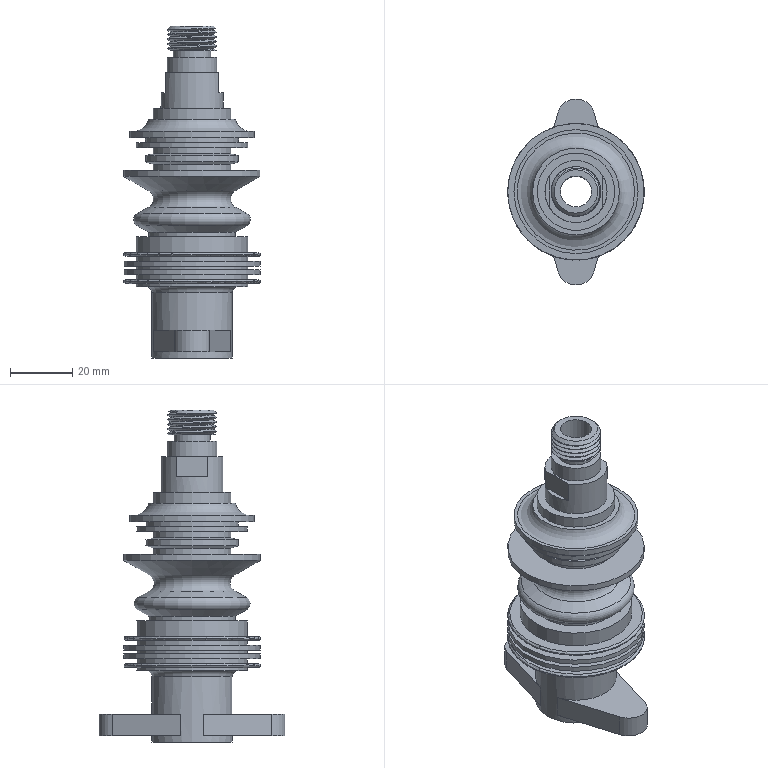Component | NX | CAMSHAFT | 1 solid | 80 faces | volume 59754 mm3 | plane 37 | cylinder 27 | torus 8 | cone 6 | spline 2 | commonest cylinder face diameters 36 x6 12 x3 44 x3 25 x3 16 x3 30 x2 26 x1 28 x1